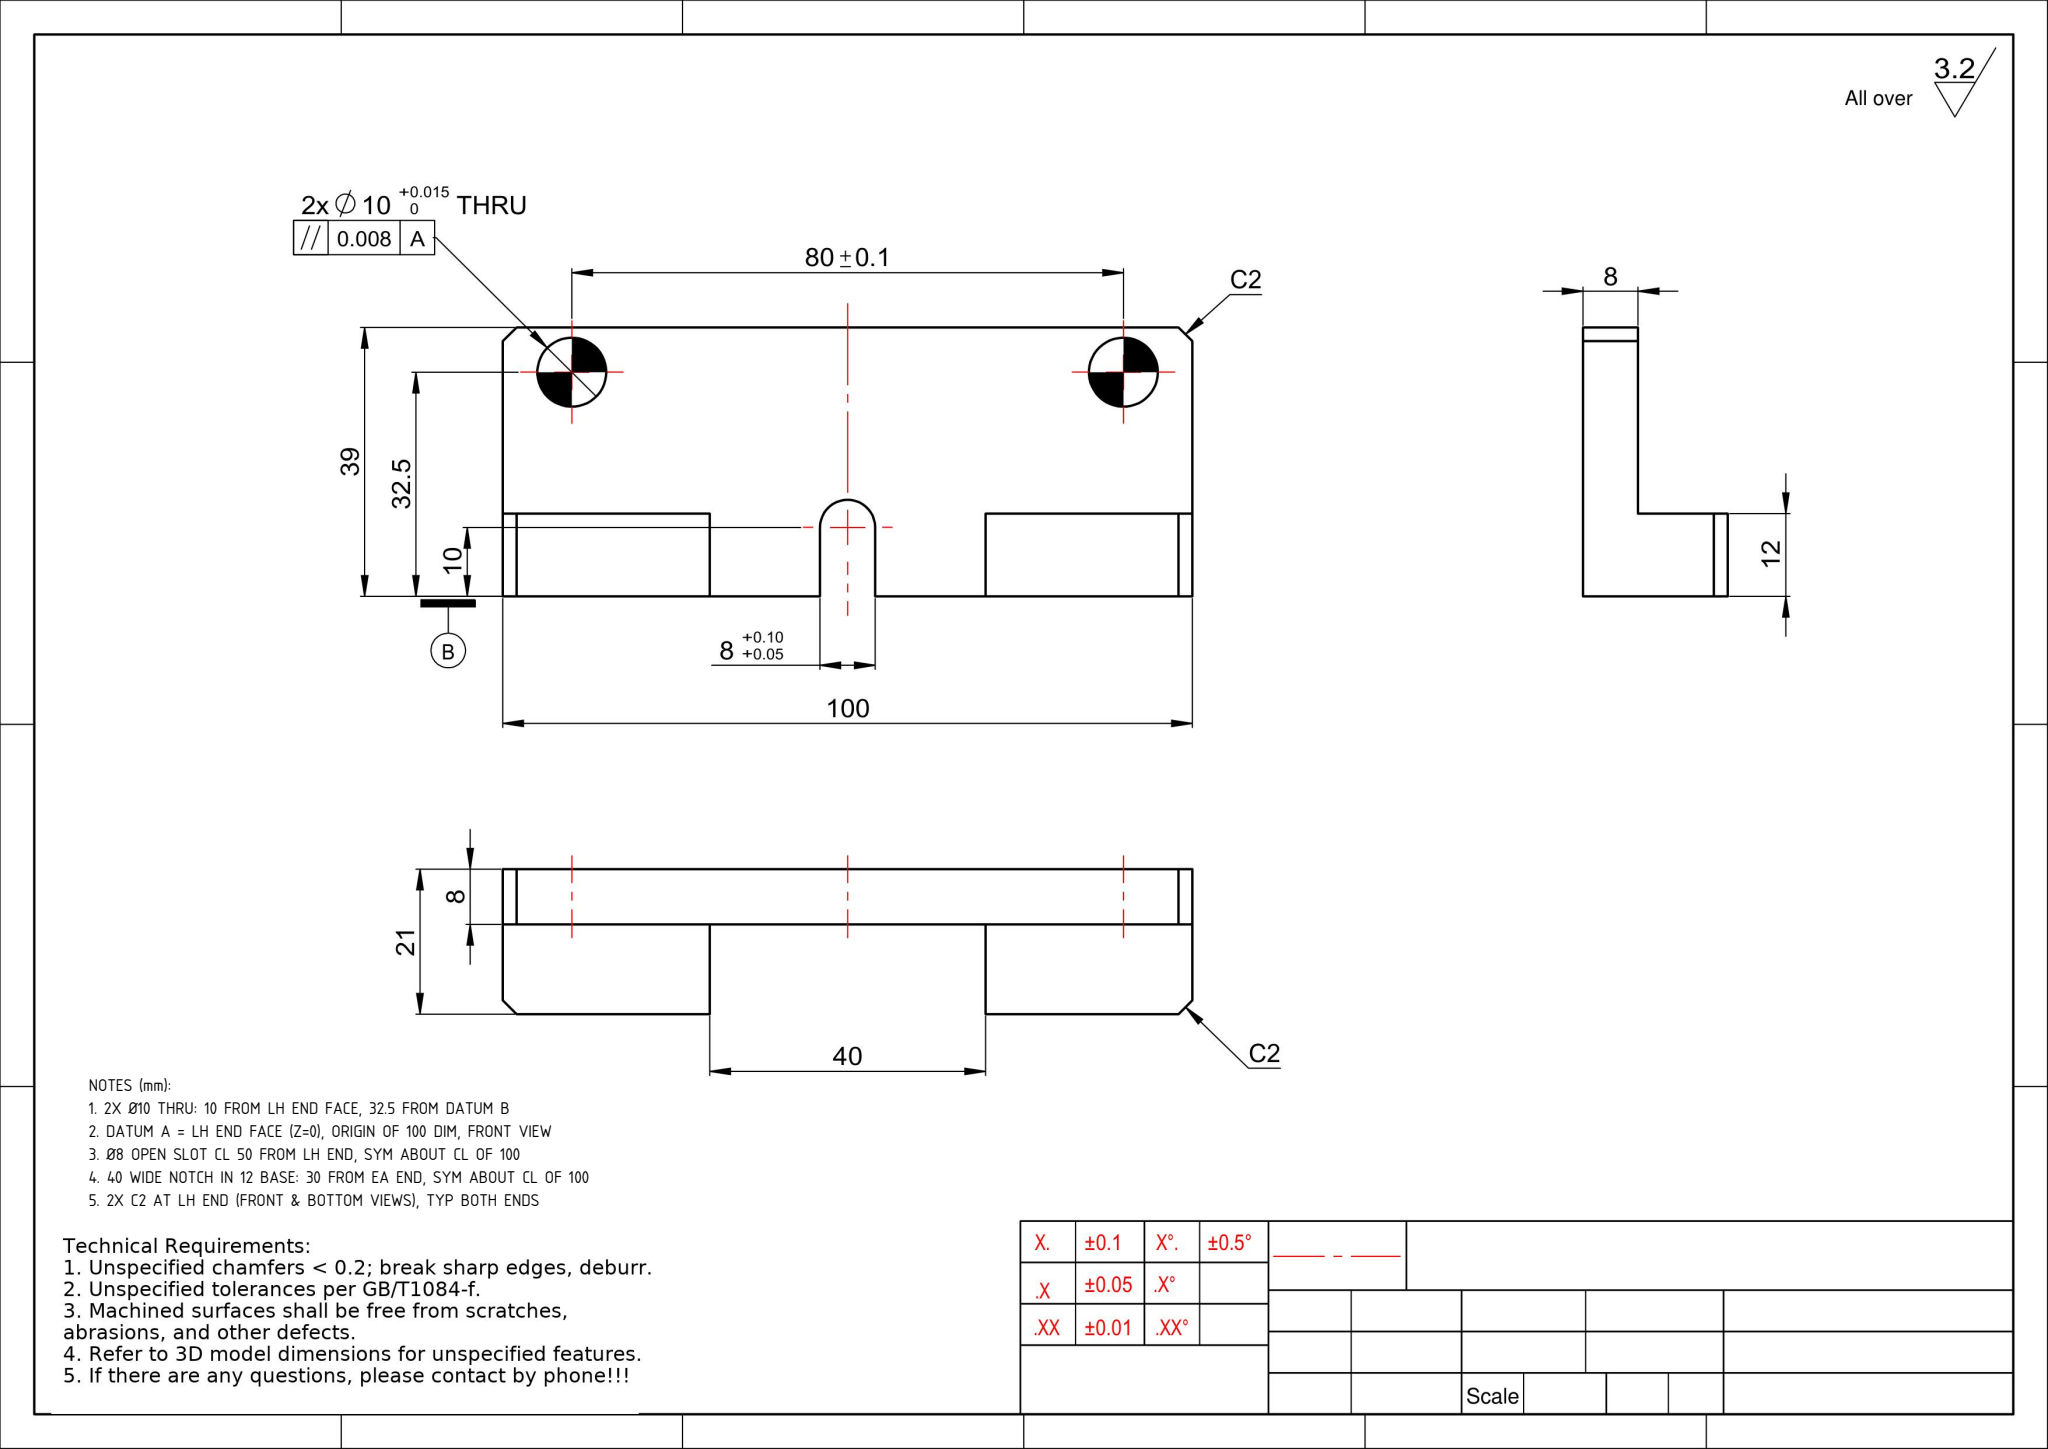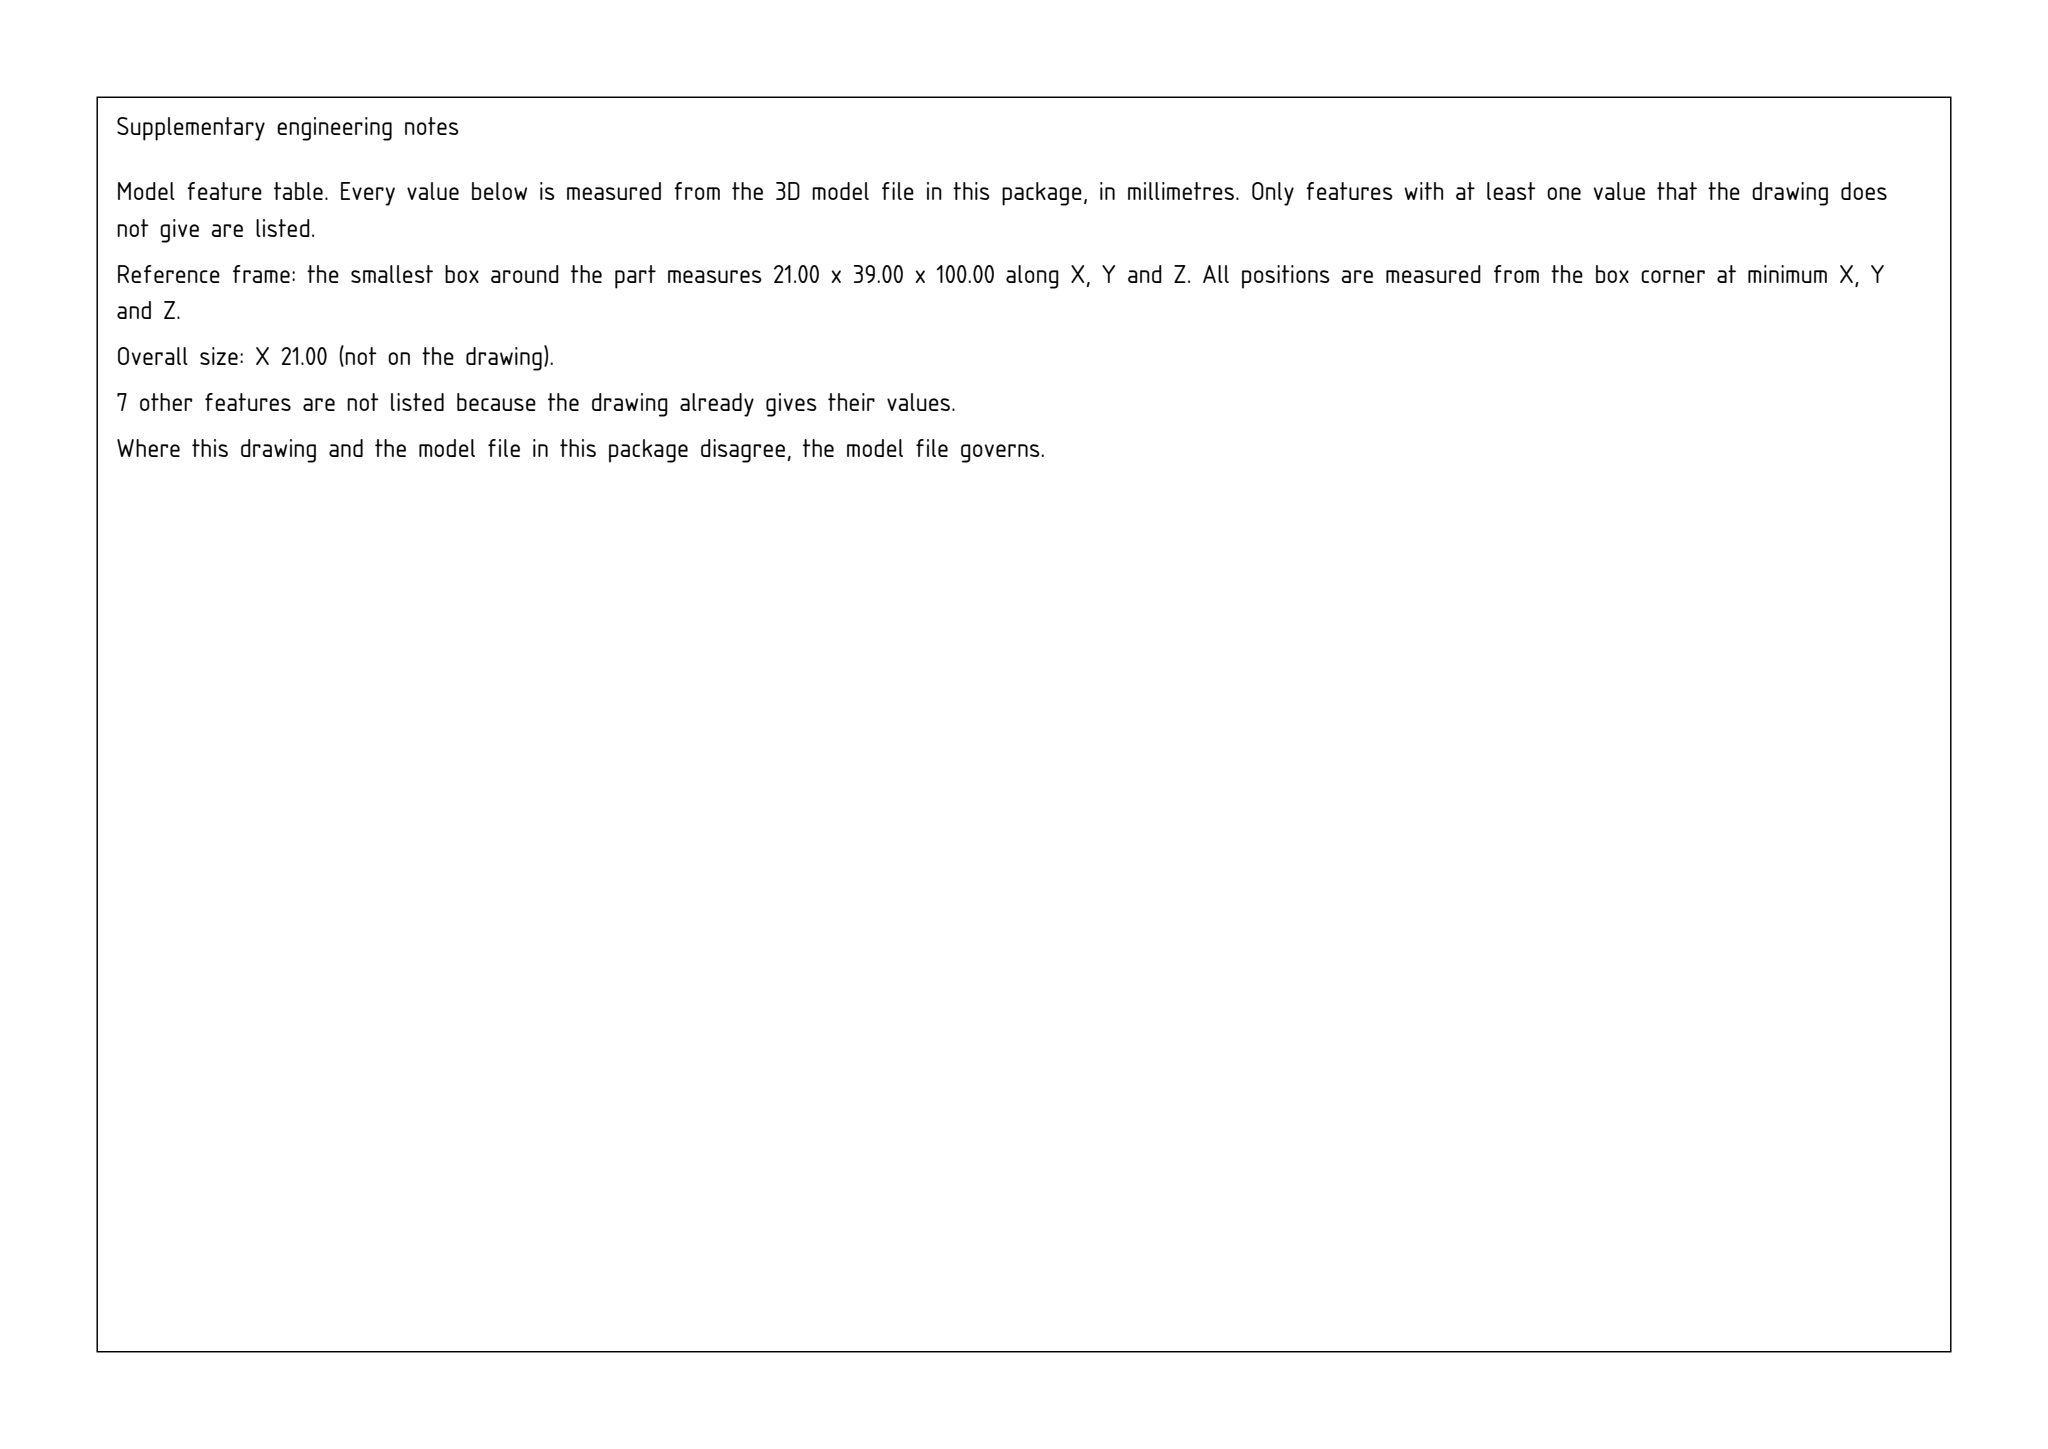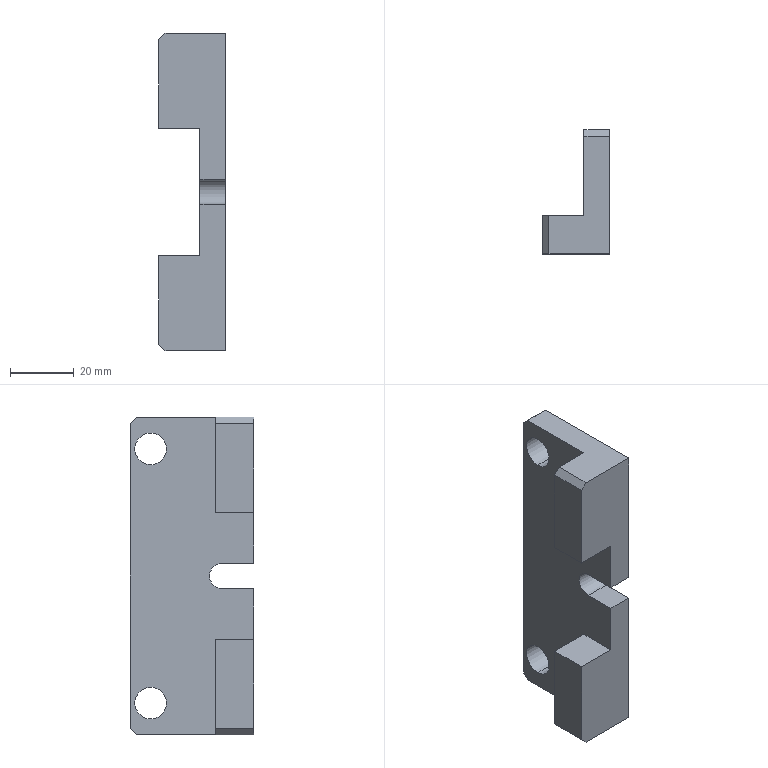Part | SolidWorks | mm | 1 solid | 24 faces | box 21 x 39 x 100 mm | volume 38382 mm3 | plane 19 | cylinder 5 | commonest cylinder face diameters 10 x4 8 x1
Drawing notes:
2X Ø10 THRU: 10 FROM LH END FACE, 32.5 FROM DATUM B | from the solid: Ø10 cylinders, axis x, at z=10 and z=90 (bbox z=100), y=32.5
DATUM A = LH END FACE (Z=0), ORIGIN OF 100 DIM, FRONT VIEW | from the solid: axis_planes z=0 end face; overall length 100 to z=100 face
Ø8 OPEN SLOT CL 50 FROM LH END, SYM ABOUT CL OF 100 | from the solid: cyl dia 8, axis x, pos z=50 of 100 length bbox
40 WIDE NOTCH IN 12 BASE: 30 FROM EA END, SYM ABOUT CL OF 100 | from the solid: z planes at 30 and 70; bbox z=100
2X C2 AT LH END (FRONT & BOTTOM VIEWS), TYP BOTH ENDS | from the solid: chamfer faces at both z ends; C2 shown at RH end only
build123d program:
from build123d import *

# Parameters (mm, degrees)
SKETCH1_W                 = 21
SKETCH1_H                 = 39
BOSS_EXTRUDE1_DEPTH       = 50
SKETCH2_W                 = 13
SKETCH2_H                 = 27
CUT_EXTRUDE1_DEPTH        = 103.423
CHAMFER1_SIZE             = 2
SIZE_MM_DOWEL_PIN_HOLE1_D = 10
SKETCH6_W                 = 13
SKETCH6_H                 = 40
CUT_EXTRUDE2_DEPTH        = 58.786
CUT_EXTRUDE3_DEPTH        = 56.22


with BuildPart() as part:
    # Sketch1 → Boss-Extrude1 (new, symmetric)
    with BuildSketch(Plane.XY):
        Rectangle(SKETCH1_W, SKETCH1_H)
    extrude(amount=BOSS_EXTRUDE1_DEPTH, both=True)

    # Sketch2 → Cut-Extrude1 (cut, through all)
    with BuildSketch(Plane.XY.offset(50)):
        with Locations((-4, 6)):
            Rectangle(SKETCH2_W, SKETCH2_H)
    extrude(amount=-CUT_EXTRUDE1_DEPTH, mode=Mode.SUBTRACT)

    # Chamfer1
    chamfer1_edges = [part.edges().sort_by_distance(p)[0] for p in [
        (-10.5, -13.5, -50),
        (-10.5, -13.5, 50),
        (6.5, 19.5, -50),
        (6.5, 19.5, 50),
    ]]
    chamfer(chamfer1_edges, length=CHAMFER1_SIZE)

    # Size mm Dowel Pin Hole1 (through all)
    with Locations(Plane.ZY.offset(-2.5)):
        with Locations((40, 13), (-40, 13)):
            Hole(SIZE_MM_DOWEL_PIN_HOLE1_D / 2)

    # Sketch6 → Cut-Extrude2 (cut, through all)
    with BuildSketch(Plane(origin=(0, -7.5, 0), x_dir=(1, 0, 0), z_dir=(0, 1, 0))):
        with Locations((-4, 0)):
            Rectangle(SKETCH6_W, SKETCH6_H)
    extrude(amount=-CUT_EXTRUDE2_DEPTH, mode=Mode.SUBTRACT)

    # Sketch7 → Cut-Extrude3 (cut, through all)
    with BuildSketch(Plane.ZY.offset(-2.5)):
        with BuildLine():
            Line((-4, -19.5), (-4, -9.5))
            ThreePointArc((-4, -9.5), (0, -5.5), (4, -9.5))
            Line((4, -9.5), (4, -19.5))
            ThreePointArc((4, -19.5), (0, -23.5), (-4, -19.5))
        make_face()
    extrude(amount=-CUT_EXTRUDE3_DEPTH, mode=Mode.SUBTRACT)


solid = part.part
STEP:
#1=CARTESIAN_POINT('',(10.5,13.,35.));
#2=VERTEX_POINT('',#1);
#3=CARTESIAN_POINT('',(10.5,13.,45.));
#4=VERTEX_POINT('',#3);
#5=CARTESIAN_POINT('',(10.5,13.,40.));
#6=DIRECTION('',(-1.,0.,0.));
#7=DIRECTION('',(0.,0.,1.));
#8=AXIS2_PLACEMENT_3D('',#5,#6,#7);
#9=CIRCLE('',#8,5.);
#10=EDGE_CURVE('',#2,#4,#9,.T.);
#11=ORIENTED_EDGE('',*,*,#10,.F.);
#12=CARTESIAN_POINT('',(2.5,13.,35.));
#13=VERTEX_POINT('',#12);
#14=CARTESIAN_POINT('',(2.5,13.,35.));
#15=DIRECTION('',(-1.,0.,0.));
#16=VECTOR('',#15,1000.);
#17=LINE('',#14,#16);
#18=EDGE_CURVE('',#2,#13,#17,.T.);
#19=ORIENTED_EDGE('',*,*,#18,.T.);
#20=CARTESIAN_POINT('',(2.5,13.,45.));
#21=VERTEX_POINT('',#20);
#22=CARTESIAN_POINT('',(2.5,13.,40.));
#23=DIRECTION('',(-1.,0.,0.));
#24=DIRECTION('',(0.,0.,1.));
#25=AXIS2_PLACEMENT_3D('',#22,#23,#24);
#26=CIRCLE('',#25,5.);
#27=EDGE_CURVE('',#13,#21,#26,.T.);
#28=ORIENTED_EDGE('',*,*,#27,.T.);
#29=CARTESIAN_POINT('',(2.5,13.,45.));
#30=DIRECTION('',(-1.,0.,0.));
#31=VECTOR('',#30,1000.);
#32=LINE('',#29,#31);
#33=EDGE_CURVE('',#4,#21,#32,.T.);
#34=ORIENTED_EDGE('',*,*,#33,.F.);
#35=EDGE_LOOP('',(#11,#19,#28,#34));
#36=FACE_OUTER_BOUND('',#35,.T.);
#37=CARTESIAN_POINT('',(2.5,13.,40.));
#38=DIRECTION('',(-1.,0.,0.));
#39=DIRECTION('',(0.,0.,1.));
#40=AXIS2_PLACEMENT_3D('',#37,#38,#39);
#41=CYLINDRICAL_SURFACE('',#40,5.);
#42=ADVANCED_FACE('',(#36),#41,.F.);
#43=CARTESIAN_POINT('',(10.5,13.,-45.));
#44=VERTEX_POINT('',#43);
#45=CARTESIAN_POINT('',(10.5,13.,-35.));
#46=VERTEX_POINT('',#45);
#47=CARTESIAN_POINT('',(10.5,13.,-40.));
#48=DIRECTION('',(-1.,0.,0.));
#49=DIRECTION('',(0.,0.,1.));
#50=AXIS2_PLACEMENT_3D('',#47,#48,#49);
#51=CIRCLE('',#50,5.);
#52=EDGE_CURVE('',#44,#46,#51,.T.);
#53=ORIENTED_EDGE('',*,*,#52,.F.);
#54=CARTESIAN_POINT('',(2.5,13.,-45.));
#55=VERTEX_POINT('',#54);
#56=CARTESIAN_POINT('',(2.5,13.,-45.));
#57=DIRECTION('',(-1.,0.,0.));
#58=VECTOR('',#57,1000.);
#59=LINE('',#56,#58);
#60=EDGE_CURVE('',#44,#55,#59,.T.);
#61=ORIENTED_EDGE('',*,*,#60,.T.);
#62=CARTESIAN_POINT('',(2.5,13.,-35.));
#63=VERTEX_POINT('',#62);
#64=CARTESIAN_POINT('',(2.5,13.,-40.));
#65=DIRECTION('',(-1.,0.,0.));
#66=DIRECTION('',(0.,0.,1.));
#67=AXIS2_PLACEMENT_3D('',#64,#65,#66);
#68=CIRCLE('',#67,5.);
#69=EDGE_CURVE('',#55,#63,#68,.T.);
#70=ORIENTED_EDGE('',*,*,#69,.T.);
#71=CARTESIAN_POINT('',(2.5,13.,-35.));
#72=DIRECTION('',(-1.,0.,0.));
#73=VECTOR('',#72,1000.);
#74=LINE('',#71,#73);
#75=EDGE_CURVE('',#46,#63,#74,.T.);
#76=ORIENTED_EDGE('',*,*,#75,.F.);
#77=EDGE_LOOP('',(#53,#61,#70,#76));
#78=FACE_OUTER_BOUND('',#77,.T.);
#79=CARTESIAN_POINT('',(2.5,13.,-40.));
#80=DIRECTION('',(-1.,0.,0.));
#81=DIRECTION('',(0.,0.,1.));
#82=AXIS2_PLACEMENT_3D('',#79,#80,#81);
#83=CYLINDRICAL_SURFACE('',#82,5.);
#84=ADVANCED_FACE('',(#78),#83,.F.);
#85=CARTESIAN_POINT('',(10.5,-19.5,-4.));
#86=VERTEX_POINT('',#85);
#87=CARTESIAN_POINT('',(10.5,-19.5,-50.));
#88=VERTEX_POINT('',#87);
#89=CARTESIAN_POINT('',(10.5,-19.5,50.));
#90=DIRECTION('',(0.,0.,-1.));
#91=VECTOR('',#90,1000.);
#92=LINE('',#89,#91);
#93=EDGE_CURVE('',#86,#88,#92,.T.);
#94=ORIENTED_EDGE('',*,*,#93,.F.);
#95=CARTESIAN_POINT('',(2.5,-19.5,-4.));
#96=VERTEX_POINT('',#95);
#97=CARTESIAN_POINT('',(10.5,-19.5,-4.));
#98=DIRECTION('',(-1.,-0.,0.));
#99=VECTOR('',#98,1000.);
#100=LINE('',#97,#99);
#101=EDGE_CURVE('',#86,#96,#100,.T.);
#102=ORIENTED_EDGE('',*,*,#101,.T.);
#103=CARTESIAN_POINT('',(2.5,-19.5,-20.));
#104=VERTEX_POINT('',#103);
#105=CARTESIAN_POINT('',(2.5,-19.5,-20.));
#106=DIRECTION('',(0.,0.,-1.));
#107=VECTOR('',#106,1000.);
#108=LINE('',#105,#107);
#109=EDGE_CURVE('',#96,#104,#108,.T.);
#110=ORIENTED_EDGE('',*,*,#109,.T.);
#111=CARTESIAN_POINT('',(-10.5,-19.5,-20.));
#112=VERTEX_POINT('',#111);
#113=CARTESIAN_POINT('',(-10.5,-19.5,-20.));
#114=DIRECTION('',(-1.,-0.,0.));
#115=VECTOR('',#114,1000.);
#116=LINE('',#113,#115);
#117=EDGE_CURVE('',#104,#112,#116,.T.);
#118=ORIENTED_EDGE('',*,*,#117,.T.);
#119=CARTESIAN_POINT('',(-10.5,-19.5,-48.));
#120=VERTEX_POINT('',#119);
#121=CARTESIAN_POINT('',(-10.5,-19.5,50.));
#122=DIRECTION('',(0.,0.,-1.));
#123=VECTOR('',#122,1000.);
#124=LINE('',#121,#123);
#125=EDGE_CURVE('',#112,#120,#124,.T.);
#126=ORIENTED_EDGE('',*,*,#125,.T.);
#127=CARTESIAN_POINT('',(-8.5,-19.5,-50.));
#128=VERTEX_POINT('',#127);
#129=CARTESIAN_POINT('',(-10.5,-19.5,-48.));
#130=DIRECTION('',(0.7071,0.,-0.7071));
#131=VECTOR('',#130,1000.);
#132=LINE('',#129,#131);
#133=EDGE_CURVE('',#120,#128,#132,.T.);
#134=ORIENTED_EDGE('',*,*,#133,.T.);
#135=CARTESIAN_POINT('',(-10.5,-19.5,-50.));
#136=DIRECTION('',(1.,0.,0.));
#137=VECTOR('',#136,1000.);
#138=LINE('',#135,#137);
#139=EDGE_CURVE('',#128,#88,#138,.T.);
#140=ORIENTED_EDGE('',*,*,#139,.T.);
#141=EDGE_LOOP('',(#94,#102,#110,#118,#126,#134,#140));
#142=FACE_OUTER_BOUND('',#141,.T.);
#143=CARTESIAN_POINT('',(-10.5,-19.5,50.));
#144=DIRECTION('',(0.,1.,0.));
#145=DIRECTION('',(0.,0.,1.));
#146=AXIS2_PLACEMENT_3D('',#143,#144,#145);
#147=PLANE('',#146);
#148=ADVANCED_FACE('',(#142),#147,.F.);
#149=ORIENTED_EDGE('',*,*,#125,.F.);
#150=CARTESIAN_POINT('',(-10.5,-7.5,-20.));
#151=VERTEX_POINT('',#150);
#152=CARTESIAN_POINT('',(-10.5,-19.5,-20.));
#153=DIRECTION('',(-0.,1.,0.));
#154=VECTOR('',#153,1000.);
#155=LINE('',#152,#154);
#156=EDGE_CURVE('',#112,#151,#155,.T.);
#157=ORIENTED_EDGE('',*,*,#156,.T.);
#158=CARTESIAN_POINT('',(-10.5,-7.5,-48.));
#159=VERTEX_POINT('',#158);
#160=CARTESIAN_POINT('',(-10.5,-7.5,-50.));
#161=DIRECTION('',(0.,0.,1.));
#162=VECTOR('',#161,1000.);
#163=LINE('',#160,#162);
#164=EDGE_CURVE('',#159,#151,#163,.T.);
#165=ORIENTED_EDGE('',*,*,#164,.F.);
#166=CARTESIAN_POINT('',(-10.5,19.5,-48.));
#167=DIRECTION('',(0.,-1.,0.));
#168=VECTOR('',#167,1000.);
#169=LINE('',#166,#168);
#170=EDGE_CURVE('',#159,#120,#169,.T.);
#171=ORIENTED_EDGE('',*,*,#170,.T.);
#172=EDGE_LOOP('',(#149,#157,#165,#171));
#173=FACE_OUTER_BOUND('',#172,.T.);
#174=CARTESIAN_POINT('',(-10.5,19.5,50.));
#175=DIRECTION('',(1.,0.,0.));
#176=DIRECTION('',(-0.,1.,0.));
#177=AXIS2_PLACEMENT_3D('',#174,#175,#176);
#178=PLANE('',#177);
#179=ADVANCED_FACE('',(#173),#178,.F.);
#180=ORIENTED_EDGE('',*,*,#164,.T.);
#181=CARTESIAN_POINT('',(2.5,-7.5,-20.));
#182=VERTEX_POINT('',#181);
#183=CARTESIAN_POINT('',(-10.5,-7.5,-20.));
#184=DIRECTION('',(-1.,-0.,0.));
#185=VECTOR('',#184,1000.);
#186=LINE('',#183,#185);
#187=EDGE_CURVE('',#182,#151,#186,.T.);
#188=ORIENTED_EDGE('',*,*,#187,.F.);
#189=CARTESIAN_POINT('',(2.5,-7.5,-50.));
#190=VERTEX_POINT('',#189);
#191=CARTESIAN_POINT('',(2.5,-7.5,-50.));
#192=DIRECTION('',(0.,0.,1.));
#193=VECTOR('',#192,1000.);
#194=LINE('',#191,#193);
#195=EDGE_CURVE('',#190,#182,#194,.T.);
#196=ORIENTED_EDGE('',*,*,#195,.F.);
#197=CARTESIAN_POINT('',(-8.5,-7.5,-50.));
#198=VERTEX_POINT('',#197);
#199=CARTESIAN_POINT('',(-10.5,-7.5,-50.));
#200=DIRECTION('',(1.,0.,0.));
#201=VECTOR('',#200,1000.);
#202=LINE('',#199,#201);
#203=EDGE_CURVE('',#198,#190,#202,.T.);
#204=ORIENTED_EDGE('',*,*,#203,.F.);
#205=CARTESIAN_POINT('',(-10.5,-7.5,-48.));
#206=DIRECTION('',(-0.7071,-0.,0.7071));
#207=VECTOR('',#206,1000.);
#208=LINE('',#205,#207);
#209=EDGE_CURVE('',#198,#159,#208,.T.);
#210=ORIENTED_EDGE('',*,*,#209,.T.);
#211=EDGE_LOOP('',(#180,#188,#196,#204,#210));
#212=FACE_OUTER_BOUND('',#211,.T.);
#213=CARTESIAN_POINT('',(-10.5,-7.5,-50.));
#214=DIRECTION('',(0.,-1.,0.));
#215=DIRECTION('',(1.,0.,0.));
#216=AXIS2_PLACEMENT_3D('',#213,#214,#215);
#217=PLANE('',#216);
#218=ADVANCED_FACE('',(#212),#217,.F.);
#219=CARTESIAN_POINT('',(10.5,13.,40.));
#220=DIRECTION('',(-1.,0.,0.));
#221=DIRECTION('',(0.,0.,1.));
#222=AXIS2_PLACEMENT_3D('',#219,#220,#221);
#223=CIRCLE('',#222,5.);
#224=EDGE_CURVE('',#4,#2,#223,.T.);
#225=ORIENTED_EDGE('',*,*,#224,.T.);
#226=ORIENTED_EDGE('',*,*,#10,.T.);
#227=EDGE_LOOP('',(#225,#226));
#228=FACE_BOUND('',#227,.T.);
#229=CARTESIAN_POINT('',(10.5,13.,-40.));
#230=DIRECTION('',(-1.,0.,0.));
#231=DIRECTION('',(0.,0.,1.));
#232=AXIS2_PLACEMENT_3D('',#229,#230,#231);
#233=CIRCLE('',#232,5.);
#234=EDGE_CURVE('',#46,#44,#233,.T.);
#235=ORIENTED_EDGE('',*,*,#234,.T.);
#236=ORIENTED_EDGE('',*,*,#52,.T.);
#237=EDGE_LOOP('',(#235,#236));
#238=FACE_BOUND('',#237,.T.);
#239=CARTESIAN_POINT('',(10.5,-9.5,4.));
#240=VERTEX_POINT('',#239);
#241=CARTESIAN_POINT('',(10.5,-9.5,-4.));
#242=VERTEX_POINT('',#241);
#243=CARTESIAN_POINT('',(10.5,-9.5,0.));
#244=DIRECTION('',(-1.,-0.,0.));
#245=DIRECTION('',(0.,-1.,0.));
#246=AXIS2_PLACEMENT_3D('',#243,#244,#245);
#247=CIRCLE('',#246,4.);
#248=EDGE_CURVE('',#240,#242,#247,.T.);
#249=ORIENTED_EDGE('',*,*,#248,.T.);
#250=CARTESIAN_POINT('',(10.5,-19.5,-4.));
#251=DIRECTION('',(0.,-1.,0.));
#252=VECTOR('',#251,1000.);
#253=LINE('',#250,#252);
#254=EDGE_CURVE('',#242,#86,#253,.T.);
#255=ORIENTED_EDGE('',*,*,#254,.T.);
#256=ORIENTED_EDGE('',*,*,#93,.T.);
#257=CARTESIAN_POINT('',(10.5,17.5,-50.));
#258=VERTEX_POINT('',#257);
#259=CARTESIAN_POINT('',(10.5,19.5,-50.));
#260=DIRECTION('',(-0.,1.,0.));
#261=VECTOR('',#260,1000.);
#262=LINE('',#259,#261);
#263=EDGE_CURVE('',#88,#258,#262,.T.);
#264=ORIENTED_EDGE('',*,*,#263,.T.);
#265=CARTESIAN_POINT('',(10.5,19.5,-48.));
#266=VERTEX_POINT('',#265);
#267=CARTESIAN_POINT('',(10.5,19.5,-48.));
#268=DIRECTION('',(-0.,0.7071,0.7071));
#269=VECTOR('',#268,1000.);
#270=LINE('',#267,#269);
#271=EDGE_CURVE('',#258,#266,#270,.T.);
#272=ORIENTED_EDGE('',*,*,#271,.T.);
#273=CARTESIAN_POINT('',(10.5,19.5,48.));
#274=VERTEX_POINT('',#273);
#275=CARTESIAN_POINT('',(10.5,19.5,50.));
#276=DIRECTION('',(0.,0.,-1.));
#277=VECTOR('',#276,1000.);
#278=LINE('',#275,#277);
#279=EDGE_CURVE('',#274,#266,#278,.T.);
#280=ORIENTED_EDGE('',*,*,#279,.F.);
#281=CARTESIAN_POINT('',(10.5,17.5,50.));
#282=VERTEX_POINT('',#281);
#283=CARTESIAN_POINT('',(10.5,17.5,50.));
#284=DIRECTION('',(0.,-0.7071,0.7071));
#285=VECTOR('',#284,1000.);
#286=LINE('',#283,#285);
#287=EDGE_CURVE('',#274,#282,#286,.T.);
#288=ORIENTED_EDGE('',*,*,#287,.T.);
#289=CARTESIAN_POINT('',(10.5,-19.5,50.));
#290=VERTEX_POINT('',#289);
#291=CARTESIAN_POINT('',(10.5,19.5,50.));
#292=DIRECTION('',(-0.,1.,0.));
#293=VECTOR('',#292,1000.);
#294=LINE('',#291,#293);
#295=EDGE_CURVE('',#290,#282,#294,.T.);
#296=ORIENTED_EDGE('',*,*,#295,.F.);
#297=CARTESIAN_POINT('',(10.5,-19.5,4.));
#298=VERTEX_POINT('',#297);
#299=CARTESIAN_POINT('',(10.5,-19.5,50.));
#300=DIRECTION('',(0.,0.,-1.));
#301=VECTOR('',#300,1000.);
#302=LINE('',#299,#301);
#303=EDGE_CURVE('',#290,#298,#302,.T.);
#304=ORIENTED_EDGE('',*,*,#303,.T.);
#305=CARTESIAN_POINT('',(10.5,-19.5,4.));
#306=DIRECTION('',(-0.,1.,0.));
#307=VECTOR('',#306,1000.);
#308=LINE('',#305,#307);
#309=EDGE_CURVE('',#298,#240,#308,.T.);
#310=ORIENTED_EDGE('',*,*,#309,.T.);
#311=EDGE_LOOP('',(#249,#255,#256,#264,#272,#280,#288,#296,#304,#310));
#312=FACE_OUTER_BOUND('',#311,.T.);
#313=CARTESIAN_POINT('',(10.5,19.5,50.));
#314=DIRECTION('',(-1.,-0.,0.));
#315=DIRECTION('',(0.,-1.,0.));
#316=AXIS2_PLACEMENT_3D('',#313,#314,#315);
#317=PLANE('',#316);
#318=ADVANCED_FACE('',(#228,#238,#312),#317,.F.);
#319=ORIENTED_EDGE('',*,*,#279,.T.);
#320=CARTESIAN_POINT('',(2.5,19.5,-48.));
#321=VERTEX_POINT('',#320);
#322=CARTESIAN_POINT('',(-10.5,19.5,-48.));
#323=DIRECTION('',(-1.,0.,0.));
#324=VECTOR('',#323,1000.);
#325=LINE('',#322,#324);
#326=EDGE_CURVE('',#266,#321,#325,.T.);
#327=ORIENTED_EDGE('',*,*,#326,.T.);
#328=CARTESIAN_POINT('',(2.5,19.5,48.));
#329=VERTEX_POINT('',#328);
#330=CARTESIAN_POINT('',(2.5,19.5,-50.));
#331=DIRECTION('',(0.,0.,1.));
#332=VECTOR('',#331,1000.);
#333=LINE('',#330,#332);
#334=EDGE_CURVE('',#321,#329,#333,.T.);
#335=ORIENTED_EDGE('',*,*,#334,.T.);
#336=CARTESIAN_POINT('',(10.5,19.5,48.));
#337=DIRECTION('',(1.,0.,0.));
#338=VECTOR('',#337,1000.);
#339=LINE('',#336,#338);
#340=EDGE_CURVE('',#329,#274,#339,.T.);
#341=ORIENTED_EDGE('',*,*,#340,.T.);
#342=EDGE_LOOP('',(#319,#327,#335,#341));
#343=FACE_OUTER_BOUND('',#342,.T.);
#344=CARTESIAN_POINT('',(-10.5,19.5,50.));
#345=DIRECTION('',(0.,-1.,0.));
#346=DIRECTION('',(0.,0.,-1.));
#347=AXIS2_PLACEMENT_3D('',#344,#345,#346);
#348=PLANE('',#347);
#349=ADVANCED_FACE('',(#343),#348,.F.);
#350=CARTESIAN_POINT('',(-10.5,-7.5,20.));
#351=VERTEX_POINT('',#350);
#352=CARTESIAN_POINT('',(-10.5,-7.5,48.));
#353=VERTEX_POINT('',#352);
#354=CARTESIAN_POINT('',(-10.5,-7.5,-50.));
#355=DIRECTION('',(0.,0.,1.));
#356=VECTOR('',#355,1000.);
#357=LINE('',#354,#356);
#358=EDGE_CURVE('',#351,#353,#357,.T.);
#359=ORIENTED_EDGE('',*,*,#358,.F.);
#360=CARTESIAN_POINT('',(-10.5,-19.5,20.));
#361=VERTEX_POINT('',#360);
#362=CARTESIAN_POINT('',(-10.5,-19.5,20.));
#363=DIRECTION('',(-0.,1.,0.));
#364=VECTOR('',#363,1000.);
#365=LINE('',#362,#364);
#366=EDGE_CURVE('',#361,#351,#365,.T.);
#367=ORIENTED_EDGE('',*,*,#366,.F.);
#368=CARTESIAN_POINT('',(-10.5,-19.5,48.));
#369=VERTEX_POINT('',#368);
#370=CARTESIAN_POINT('',(-10.5,-19.5,50.));
#371=DIRECTION('',(0.,0.,-1.));
#372=VECTOR('',#371,1000.);
#373=LINE('',#370,#372);
#374=EDGE_CURVE('',#369,#361,#373,.T.);
#375=ORIENTED_EDGE('',*,*,#374,.F.);
#376=CARTESIAN_POINT('',(-10.5,-7.5,48.));
#377=DIRECTION('',(-0.,1.,0.));
#378=VECTOR('',#377,1000.);
#379=LINE('',#376,#378);
#380=EDGE_CURVE('',#369,#353,#379,.T.);
#381=ORIENTED_EDGE('',*,*,#380,.T.);
#382=EDGE_LOOP('',(#359,#367,#375,#381));
#383=FACE_OUTER_BOUND('',#382,.T.);
#384=CARTESIAN_POINT('',(-10.5,19.5,50.));
#385=DIRECTION('',(1.,0.,0.));
#386=DIRECTION('',(-0.,1.,0.));
#387=AXIS2_PLACEMENT_3D('',#384,#385,#386);
#388=PLANE('',#387);
#389=ADVANCED_FACE('',(#383),#388,.F.);
#390=CARTESIAN_POINT('',(2.5,-19.5,20.));
#391=VERTEX_POINT('',#390);
#392=CARTESIAN_POINT('',(2.5,-19.5,4.));
#393=VERTEX_POINT('',#392);
#394=CARTESIAN_POINT('',(2.5,-19.5,-20.));
#395=DIRECTION('',(0.,0.,-1.));
#396=VECTOR('',#395,1000.);
#397=LINE('',#394,#396);
#398=EDGE_CURVE('',#391,#393,#397,.T.);
#399=ORIENTED_EDGE('',*,*,#398,.T.);
#400=CARTESIAN_POINT('',(10.5,-19.5,4.));
#401=DIRECTION('',(-1.,-0.,0.));
#402=VECTOR('',#401,1000.);
#403=LINE('',#400,#402);
#404=EDGE_CURVE('',#298,#393,#403,.T.);
#405=ORIENTED_EDGE('',*,*,#404,.F.);
#406=ORIENTED_EDGE('',*,*,#303,.F.);
#407=CARTESIAN_POINT('',(-8.5,-19.5,50.));
#408=VERTEX_POINT('',#407);
#409=CARTESIAN_POINT('',(-10.5,-19.5,50.));
#410=DIRECTION('',(1.,0.,0.));
#411=VECTOR('',#410,1000.);
#412=LINE('',#409,#411);
#413=EDGE_CURVE('',#408,#290,#412,.T.);
#414=ORIENTED_EDGE('',*,*,#413,.F.);
#415=CARTESIAN_POINT('',(-8.5,-19.5,50.));
#416=DIRECTION('',(-0.7071,0.,-0.7071));
#417=VECTOR('',#416,1000.);
#418=LINE('',#415,#417);
#419=EDGE_CURVE('',#408,#369,#418,.T.);
#420=ORIENTED_EDGE('',*,*,#419,.T.);
#421=ORIENTED_EDGE('',*,*,#374,.T.);
#422=CARTESIAN_POINT('',(-10.5,-19.5,20.));
#423=DIRECTION('',(1.,0.,0.));
#424=VECTOR('',#423,1000.);
#425=LINE('',#422,#424);
#426=EDGE_CURVE('',#361,#391,#425,.T.);
#427=ORIENTED_EDGE('',*,*,#426,.T.);
#428=EDGE_LOOP('',(#399,#405,#406,#414,#420,#421,#427));
#429=FACE_OUTER_BOUND('',#428,.T.);
#430=CARTESIAN_POINT('',(-10.5,-19.5,50.));
#431=DIRECTION('',(0.,1.,0.));
#432=DIRECTION('',(0.,0.,1.));
#433=AXIS2_PLACEMENT_3D('',#430,#431,#432);
#434=PLANE('',#433);
#435=ADVANCED_FACE('',(#429),#434,.F.);
#436=ORIENTED_EDGE('',*,*,#295,.T.);
#437=CARTESIAN_POINT('',(2.5,17.5,50.));
#438=VERTEX_POINT('',#437);
#439=CARTESIAN_POINT('',(2.5,17.5,50.));
#440=DIRECTION('',(-1.,0.,0.));
#441=VECTOR('',#440,1000.);
#442=LINE('',#439,#441);
#443=EDGE_CURVE('',#282,#438,#442,.T.);
#444=ORIENTED_EDGE('',*,*,#443,.T.);
#445=CARTESIAN_POINT('',(2.5,-7.5,50.));
#446=VERTEX_POINT('',#445);
#447=CARTESIAN_POINT('',(2.5,19.5,50.));
#448=DIRECTION('',(-0.,1.,0.));
#449=VECTOR('',#448,1000.);
#450=LINE('',#447,#449);
#451=EDGE_CURVE('',#446,#438,#450,.T.);
#452=ORIENTED_EDGE('',*,*,#451,.F.);
#453=CARTESIAN_POINT('',(-8.5,-7.5,50.));
#454=VERTEX_POINT('',#453);
#455=CARTESIAN_POINT('',(-10.5,-7.5,50.));
#456=DIRECTION('',(1.,0.,0.));
#457=VECTOR('',#456,1000.);
#458=LINE('',#455,#457);
#459=EDGE_CURVE('',#454,#446,#458,.T.);
#460=ORIENTED_EDGE('',*,*,#459,.F.);
#461=CARTESIAN_POINT('',(-8.5,-19.5,50.));
#462=DIRECTION('',(0.,-1.,0.));
#463=VECTOR('',#462,1000.);
#464=LINE('',#461,#463);
#465=EDGE_CURVE('',#454,#408,#464,.T.);
#466=ORIENTED_EDGE('',*,*,#465,.T.);
#467=ORIENTED_EDGE('',*,*,#413,.T.);
#468=EDGE_LOOP('',(#436,#444,#452,#460,#466,#467));
#469=FACE_OUTER_BOUND('',#468,.T.);
#470=CARTESIAN_POINT('',(0.,0.,50.));
#471=DIRECTION('',(0.,0.,1.));
#472=DIRECTION('',(1.,0.,0.));
#473=AXIS2_PLACEMENT_3D('',#470,#471,#472);
#474=PLANE('',#473);
#475=ADVANCED_FACE('',(#469),#474,.T.);
#476=CARTESIAN_POINT('',(2.5,17.5,-50.));
#477=VERTEX_POINT('',#476);
#478=CARTESIAN_POINT('',(2.5,19.5,-50.));
#479=DIRECTION('',(-0.,1.,0.));
#480=VECTOR('',#479,1000.);
#481=LINE('',#478,#480);
#482=EDGE_CURVE('',#190,#477,#481,.T.);
#483=ORIENTED_EDGE('',*,*,#482,.T.);
#484=CARTESIAN_POINT('',(0.,17.5,-50.));
#485=DIRECTION('',(1.,0.,0.));
#486=VECTOR('',#485,1000.);
#487=LINE('',#484,#486);
#488=EDGE_CURVE('',#477,#258,#487,.T.);
#489=ORIENTED_EDGE('',*,*,#488,.T.);
#490=ORIENTED_EDGE('',*,*,#263,.F.);
#491=ORIENTED_EDGE('',*,*,#139,.F.);
#492=CARTESIAN_POINT('',(-8.5,-0.,-50.));
#493=DIRECTION('',(-0.,1.,0.));
#494=VECTOR('',#493,1000.);
#495=LINE('',#492,#494);
#496=EDGE_CURVE('',#128,#198,#495,.T.);
#497=ORIENTED_EDGE('',*,*,#496,.T.);
#498=ORIENTED_EDGE('',*,*,#203,.T.);
#499=EDGE_LOOP('',(#483,#489,#490,#491,#497,#498));
#500=FACE_OUTER_BOUND('',#499,.T.);
#501=CARTESIAN_POINT('',(0.,0.,-50.));
#502=DIRECTION('',(0.,0.,1.));
#503=DIRECTION('',(1.,0.,0.));
#504=AXIS2_PLACEMENT_3D('',#501,#502,#503);
#505=PLANE('',#504);
#506=ADVANCED_FACE('',(#500),#505,.F.);
#507=CARTESIAN_POINT('',(2.5,13.,40.));
#508=DIRECTION('',(-1.,0.,0.));
#509=DIRECTION('',(0.,0.,1.));
#510=AXIS2_PLACEMENT_3D('',#507,#508,#509);
#511=CIRCLE('',#510,5.);
#512=EDGE_CURVE('',#21,#13,#511,.T.);
#513=ORIENTED_EDGE('',*,*,#512,.F.);
#514=ORIENTED_EDGE('',*,*,#27,.F.);
#515=EDGE_LOOP('',(#513,#514));
#516=FACE_BOUND('',#515,.T.);
#517=CARTESIAN_POINT('',(2.5,13.,-40.));
#518=DIRECTION('',(-1.,0.,0.));
#519=DIRECTION('',(0.,0.,1.));
#520=AXIS2_PLACEMENT_3D('',#517,#518,#519);
#521=CIRCLE('',#520,5.);
#522=EDGE_CURVE('',#63,#55,#521,.T.);
#523=ORIENTED_EDGE('',*,*,#522,.F.);
#524=ORIENTED_EDGE('',*,*,#69,.F.);
#525=EDGE_LOOP('',(#523,#524));
#526=FACE_BOUND('',#525,.T.);
#527=ORIENTED_EDGE('',*,*,#109,.F.);
#528=CARTESIAN_POINT('',(2.5,-9.5,-4.));
#529=VERTEX_POINT('',#528);
#530=CARTESIAN_POINT('',(2.5,-19.5,-4.));
#531=DIRECTION('',(0.,-1.,0.));
#532=VECTOR('',#531,1000.);
#533=LINE('',#530,#532);
#534=EDGE_CURVE('',#529,#96,#533,.T.);
#535=ORIENTED_EDGE('',*,*,#534,.F.);
#536=CARTESIAN_POINT('',(2.5,-9.5,4.));
#537=VERTEX_POINT('',#536);
#538=CARTESIAN_POINT('',(2.5,-9.5,0.));
#539=DIRECTION('',(-1.,-0.,0.));
#540=DIRECTION('',(0.,-1.,0.));
#541=AXIS2_PLACEMENT_3D('',#538,#539,#540);
#542=CIRCLE('',#541,4.);
#543=EDGE_CURVE('',#537,#529,#542,.T.);
#544=ORIENTED_EDGE('',*,*,#543,.F.);
#545=CARTESIAN_POINT('',(2.5,-19.5,4.));
#546=DIRECTION('',(-0.,1.,0.));
#547=VECTOR('',#546,1000.);
#548=LINE('',#545,#547);
#549=EDGE_CURVE('',#393,#537,#548,.T.);
#550=ORIENTED_EDGE('',*,*,#549,.F.);
#551=ORIENTED_EDGE('',*,*,#398,.F.);
#552=CARTESIAN_POINT('',(2.5,-7.5,20.));
#553=VERTEX_POINT('',#552);
#554=CARTESIAN_POINT('',(2.5,-19.5,20.));
#555=DIRECTION('',(-0.,1.,0.));
#556=VECTOR('',#555,1000.);
#557=LINE('',#554,#556);
#558=EDGE_CURVE('',#391,#553,#557,.T.);
#559=ORIENTED_EDGE('',*,*,#558,.T.);
#560=CARTESIAN_POINT('',(2.5,-7.5,-50.));
#561=DIRECTION('',(0.,0.,1.));
#562=VECTOR('',#561,1000.);
#563=LINE('',#560,#562);
#564=EDGE_CURVE('',#553,#446,#563,.T.);
#565=ORIENTED_EDGE('',*,*,#564,.T.);
#566=ORIENTED_EDGE('',*,*,#451,.T.);
#567=CARTESIAN_POINT('',(2.5,17.5,50.));
#568=DIRECTION('',(-0.,0.7071,-0.7071));
#569=VECTOR('',#568,1000.);
#570=LINE('',#567,#569);
#571=EDGE_CURVE('',#438,#329,#570,.T.);
#572=ORIENTED_EDGE('',*,*,#571,.T.);
#573=ORIENTED_EDGE('',*,*,#334,.F.);
#574=CARTESIAN_POINT('',(2.5,19.5,-48.));
#575=DIRECTION('',(0.,-0.7071,-0.7071));
#576=VECTOR('',#575,1000.);
#577=LINE('',#574,#576);
#578=EDGE_CURVE('',#321,#477,#577,.T.);
#579=ORIENTED_EDGE('',*,*,#578,.T.);
#580=ORIENTED_EDGE('',*,*,#482,.F.);
#581=ORIENTED_EDGE('',*,*,#195,.T.);
#582=CARTESIAN_POINT('',(2.5,-19.5,-20.));
#583=DIRECTION('',(-0.,1.,0.));
#584=VECTOR('',#583,1000.);
#585=LINE('',#582,#584);
#586=EDGE_CURVE('',#104,#182,#585,.T.);
#587=ORIENTED_EDGE('',*,*,#586,.F.);
#588=EDGE_LOOP('',(#527,#535,#544,#550,#551,#559,#565,#566,#572,#573,#579,#580,#581,#587));
#589=FACE_OUTER_BOUND('',#588,.T.);
#590=CARTESIAN_POINT('',(2.5,19.5,-50.));
#591=DIRECTION('',(1.,0.,0.));
#592=DIRECTION('',(-0.,1.,0.));
#593=AXIS2_PLACEMENT_3D('',#590,#591,#592);
#594=PLANE('',#593);
#595=ADVANCED_FACE('',(#516,#526,#589),#594,.F.);
#596=ORIENTED_EDGE('',*,*,#564,.F.);
#597=CARTESIAN_POINT('',(-10.5,-7.5,20.));
#598=DIRECTION('',(1.,0.,0.));
#599=VECTOR('',#598,1000.);
#600=LINE('',#597,#599);
#601=EDGE_CURVE('',#351,#553,#600,.T.);
#602=ORIENTED_EDGE('',*,*,#601,.F.);
#603=ORIENTED_EDGE('',*,*,#358,.T.);
#604=CARTESIAN_POINT('',(-8.5,-7.5,50.));
#605=DIRECTION('',(0.7071,0.,0.7071));
#606=VECTOR('',#605,1000.);
#607=LINE('',#604,#606);
#608=EDGE_CURVE('',#353,#454,#607,.T.);
#609=ORIENTED_EDGE('',*,*,#608,.T.);
#610=ORIENTED_EDGE('',*,*,#459,.T.);
#611=EDGE_LOOP('',(#596,#602,#603,#609,#610));
#612=FACE_OUTER_BOUND('',#611,.T.);
#613=CARTESIAN_POINT('',(-10.5,-7.5,-50.));
#614=DIRECTION('',(0.,-1.,0.));
#615=DIRECTION('',(1.,0.,0.));
#616=AXIS2_PLACEMENT_3D('',#613,#614,#615);
#617=PLANE('',#616);
#618=ADVANCED_FACE('',(#612),#617,.F.);
#619=ORIENTED_EDGE('',*,*,#271,.F.);
#620=ORIENTED_EDGE('',*,*,#488,.F.);
#621=ORIENTED_EDGE('',*,*,#578,.F.);
#622=ORIENTED_EDGE('',*,*,#326,.F.);
#623=EDGE_LOOP('',(#619,#620,#621,#622));
#624=FACE_OUTER_BOUND('',#623,.T.);
#625=CARTESIAN_POINT('',(-10.5,19.5,-48.));
#626=DIRECTION('',(0.,-0.7071,0.7071));
#627=DIRECTION('',(-1.,0.,0.));
#628=AXIS2_PLACEMENT_3D('',#625,#626,#627);
#629=PLANE('',#628);
#630=ADVANCED_FACE('',(#624),#629,.F.);
#631=ORIENTED_EDGE('',*,*,#287,.F.);
#632=ORIENTED_EDGE('',*,*,#340,.F.);
#633=ORIENTED_EDGE('',*,*,#571,.F.);
#634=ORIENTED_EDGE('',*,*,#443,.F.);
#635=EDGE_LOOP('',(#631,#632,#633,#634));
#636=FACE_OUTER_BOUND('',#635,.T.);
#637=CARTESIAN_POINT('',(0.,17.5,50.));
#638=DIRECTION('',(0.,0.7071,0.7071));
#639=DIRECTION('',(1.,0.,0.));
#640=AXIS2_PLACEMENT_3D('',#637,#638,#639);
#641=PLANE('',#640);
#642=ADVANCED_FACE('',(#636),#641,.T.);
#643=ORIENTED_EDGE('',*,*,#608,.F.);
#644=ORIENTED_EDGE('',*,*,#380,.F.);
#645=ORIENTED_EDGE('',*,*,#419,.F.);
#646=ORIENTED_EDGE('',*,*,#465,.F.);
#647=EDGE_LOOP('',(#643,#644,#645,#646));
#648=FACE_OUTER_BOUND('',#647,.T.);
#649=CARTESIAN_POINT('',(-8.5,-0.,50.));
#650=DIRECTION('',(-0.7071,-0.,0.7071));
#651=DIRECTION('',(-0.,1.,0.));
#652=AXIS2_PLACEMENT_3D('',#649,#650,#651);
#653=PLANE('',#652);
#654=ADVANCED_FACE('',(#648),#653,.T.);
#655=ORIENTED_EDGE('',*,*,#209,.F.);
#656=ORIENTED_EDGE('',*,*,#496,.F.);
#657=ORIENTED_EDGE('',*,*,#133,.F.);
#658=ORIENTED_EDGE('',*,*,#170,.F.);
#659=EDGE_LOOP('',(#655,#656,#657,#658));
#660=FACE_OUTER_BOUND('',#659,.T.);
#661=CARTESIAN_POINT('',(-10.5,19.5,-48.));
#662=DIRECTION('',(0.7071,0.,0.7071));
#663=DIRECTION('',(0.,-1.,0.));
#664=AXIS2_PLACEMENT_3D('',#661,#662,#663);
#665=PLANE('',#664);
#666=ADVANCED_FACE('',(#660),#665,.F.);
#667=ORIENTED_EDGE('',*,*,#60,.F.);
#668=ORIENTED_EDGE('',*,*,#234,.F.);
#669=ORIENTED_EDGE('',*,*,#75,.T.);
#670=ORIENTED_EDGE('',*,*,#522,.T.);
#671=EDGE_LOOP('',(#667,#668,#669,#670));
#672=FACE_OUTER_BOUND('',#671,.T.);
#673=CARTESIAN_POINT('',(2.5,13.,-40.));
#674=DIRECTION('',(-1.,0.,0.));
#675=DIRECTION('',(0.,0.,1.));
#676=AXIS2_PLACEMENT_3D('',#673,#674,#675);
#677=CYLINDRICAL_SURFACE('',#676,5.);
#678=ADVANCED_FACE('',(#672),#677,.F.);
#679=ORIENTED_EDGE('',*,*,#18,.F.);
#680=ORIENTED_EDGE('',*,*,#224,.F.);
#681=ORIENTED_EDGE('',*,*,#33,.T.);
#682=ORIENTED_EDGE('',*,*,#512,.T.);
#683=EDGE_LOOP('',(#679,#680,#681,#682));
#684=FACE_OUTER_BOUND('',#683,.T.);
#685=CARTESIAN_POINT('',(2.5,13.,40.));
#686=DIRECTION('',(-1.,0.,0.));
#687=DIRECTION('',(0.,0.,1.));
#688=AXIS2_PLACEMENT_3D('',#685,#686,#687);
#689=CYLINDRICAL_SURFACE('',#688,5.);
#690=ADVANCED_FACE('',(#684),#689,.F.);
#691=ORIENTED_EDGE('',*,*,#187,.T.);
#692=ORIENTED_EDGE('',*,*,#156,.F.);
#693=ORIENTED_EDGE('',*,*,#117,.F.);
#694=ORIENTED_EDGE('',*,*,#586,.T.);
#695=EDGE_LOOP('',(#691,#692,#693,#694));
#696=FACE_OUTER_BOUND('',#695,.T.);
#697=CARTESIAN_POINT('',(-10.5,-19.5,-20.));
#698=DIRECTION('',(-0.,-0.,-1.));
#699=DIRECTION('',(-1.,0.,0.));
#700=AXIS2_PLACEMENT_3D('',#697,#698,#699);
#701=PLANE('',#700);
#702=ADVANCED_FACE('',(#696),#701,.F.);
#703=ORIENTED_EDGE('',*,*,#601,.T.);
#704=ORIENTED_EDGE('',*,*,#558,.F.);
#705=ORIENTED_EDGE('',*,*,#426,.F.);
#706=ORIENTED_EDGE('',*,*,#366,.T.);
#707=EDGE_LOOP('',(#703,#704,#705,#706));
#708=FACE_OUTER_BOUND('',#707,.T.);
#709=CARTESIAN_POINT('',(-10.5,-19.5,20.));
#710=DIRECTION('',(-0.,-0.,1.));
#711=DIRECTION('',(1.,0.,0.));
#712=AXIS2_PLACEMENT_3D('',#709,#710,#711);
#713=PLANE('',#712);
#714=ADVANCED_FACE('',(#708),#713,.F.);
#715=ORIENTED_EDGE('',*,*,#534,.T.);
#716=ORIENTED_EDGE('',*,*,#101,.F.);
#717=ORIENTED_EDGE('',*,*,#254,.F.);
#718=CARTESIAN_POINT('',(10.5,-9.5,-4.));
#719=DIRECTION('',(-1.,-0.,0.));
#720=VECTOR('',#719,1000.);
#721=LINE('',#718,#720);
#722=EDGE_CURVE('',#242,#529,#721,.T.);
#723=ORIENTED_EDGE('',*,*,#722,.T.);
#724=EDGE_LOOP('',(#715,#716,#717,#723));
#725=FACE_OUTER_BOUND('',#724,.T.);
#726=CARTESIAN_POINT('',(10.5,-19.5,-4.));
#727=DIRECTION('',(0.,-0.,-1.));
#728=DIRECTION('',(0.,1.,-0.));
#729=AXIS2_PLACEMENT_3D('',#726,#727,#728);
#730=PLANE('',#729);
#731=ADVANCED_FACE('',(#725),#730,.F.);
#732=ORIENTED_EDGE('',*,*,#543,.T.);
#733=ORIENTED_EDGE('',*,*,#722,.F.);
#734=ORIENTED_EDGE('',*,*,#248,.F.);
#735=CARTESIAN_POINT('',(10.5,-9.5,4.));
#736=DIRECTION('',(-1.,-0.,0.));
#737=VECTOR('',#736,1000.);
#738=LINE('',#735,#737);
#739=EDGE_CURVE('',#240,#537,#738,.T.);
#740=ORIENTED_EDGE('',*,*,#739,.T.);
#741=EDGE_LOOP('',(#732,#733,#734,#740));
#742=FACE_OUTER_BOUND('',#741,.T.);
#743=CARTESIAN_POINT('',(10.5,-9.5,0.));
#744=DIRECTION('',(-1.,-0.,0.));
#745=DIRECTION('',(0.,-1.,0.));
#746=AXIS2_PLACEMENT_3D('',#743,#744,#745);
#747=CYLINDRICAL_SURFACE('',#746,4.);
#748=ADVANCED_FACE('',(#742),#747,.F.);
#749=ORIENTED_EDGE('',*,*,#549,.T.);
#750=ORIENTED_EDGE('',*,*,#739,.F.);
#751=ORIENTED_EDGE('',*,*,#309,.F.);
#752=ORIENTED_EDGE('',*,*,#404,.T.);
#753=EDGE_LOOP('',(#749,#750,#751,#752));
#754=FACE_OUTER_BOUND('',#753,.T.);
#755=CARTESIAN_POINT('',(10.5,-19.5,4.));
#756=DIRECTION('',(0.,-0.,1.));
#757=DIRECTION('',(0.,-1.,-0.));
#758=AXIS2_PLACEMENT_3D('',#755,#756,#757);
#759=PLANE('',#758);
#760=ADVANCED_FACE('',(#754),#759,.F.);
#761=CLOSED_SHELL('',(#42,#84,#148,#179,#218,#318,#349,#389,#435,#475,#506,#595,#618,#630,#642,#654,#666,#678,#690,#702,#714,#731,#748,#760));
#762=MANIFOLD_SOLID_BREP('',#761);
#763=CARTESIAN_POINT('',(0.,0.,0.));
#764=DIRECTION('',(0.,0.,1.));
#765=DIRECTION('',(1.,0.,0.));
#766=AXIS2_PLACEMENT_3D('',#763,#764,#765);
#767=(LENGTH_UNIT()NAMED_UNIT(*)SI_UNIT(.MILLI.,.METRE.));
#768=UNCERTAINTY_MEASURE_WITH_UNIT(LENGTH_MEASURE(0.00001),#767,'','');
#769=(NAMED_UNIT(*)PLANE_ANGLE_UNIT()SI_UNIT($,.RADIAN.));
#770=(NAMED_UNIT(*)SI_UNIT($,.STERADIAN.)SOLID_ANGLE_UNIT());
#771=(GEOMETRIC_REPRESENTATION_CONTEXT(3)GLOBAL_UNCERTAINTY_ASSIGNED_CONTEXT((#768))GLOBAL_UNIT_ASSIGNED_CONTEXT((#767,#769,#770))REPRESENTATION_CONTEXT('',''));
#772=ADVANCED_BREP_SHAPE_REPRESENTATION('',(#762,#766),#771);